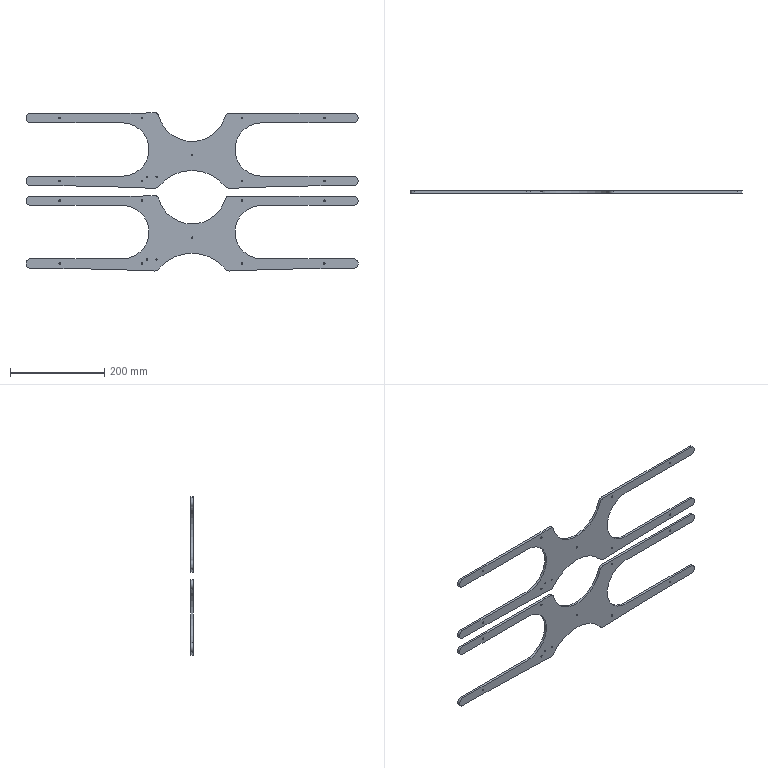CAM job | Mastercam | mm | 4 operations | part box 703 x 5 x 334.52
1. Contour (Ramp) | 3 - 3 平铣刀
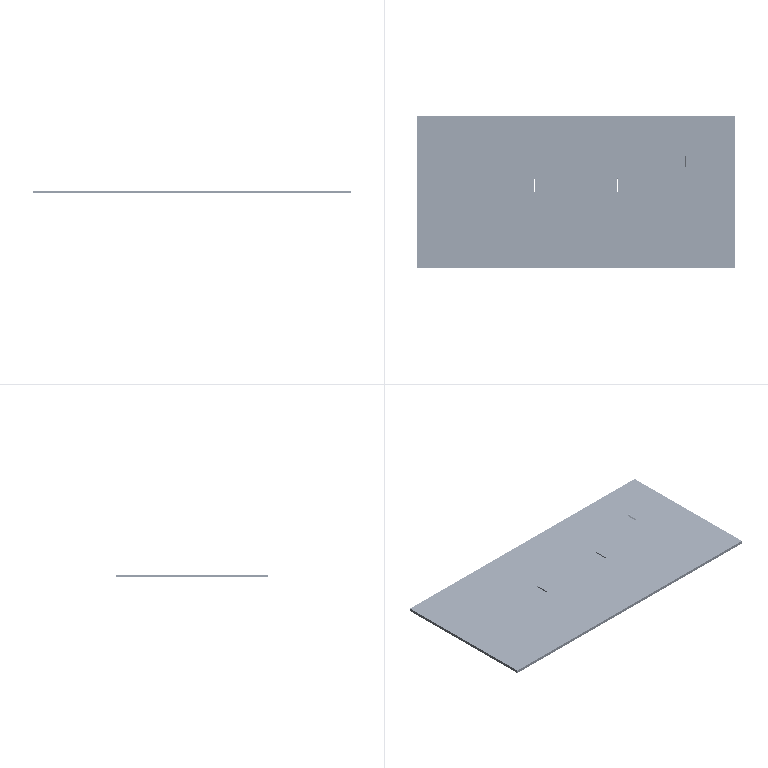2. Contour (2D) | 3 - 3 平铣刀
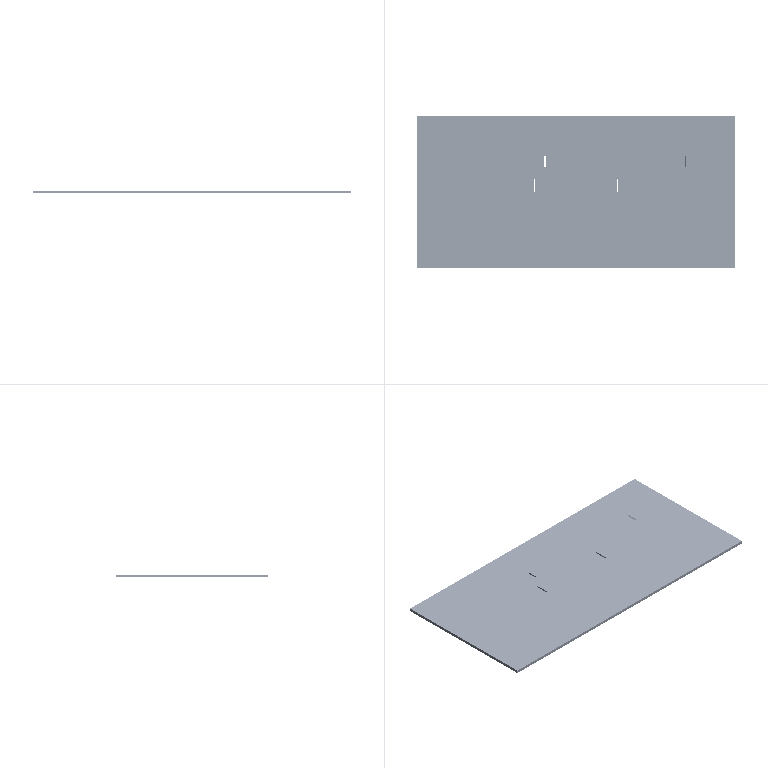3. Drill/Counterbore | 7 - 4 倒角刀
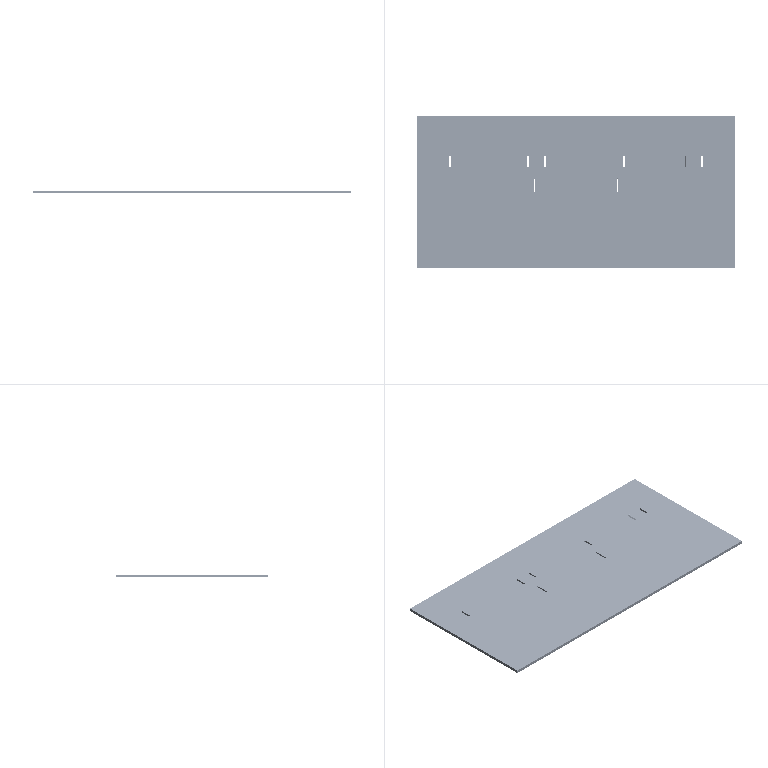4. Contour (2D chamfer) | 7 - 4 倒角刀